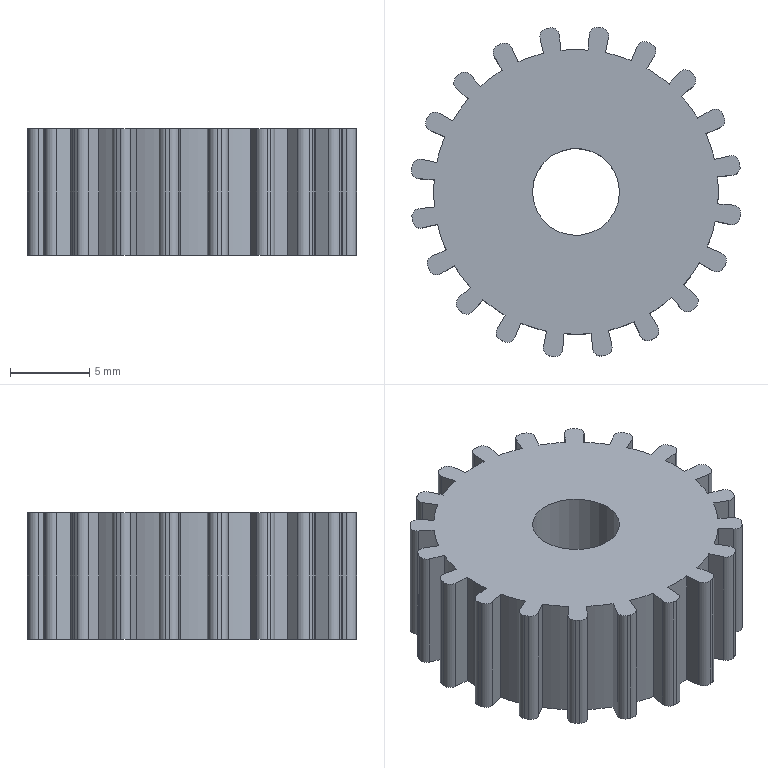Component | NX | GEAR | 1 solid | 123 faces | volume 2117 mm3 | cylinder 81 | plane 42 | commonest cylinder face diameters 1 x40 21 x20 18 x20 5.5 x1